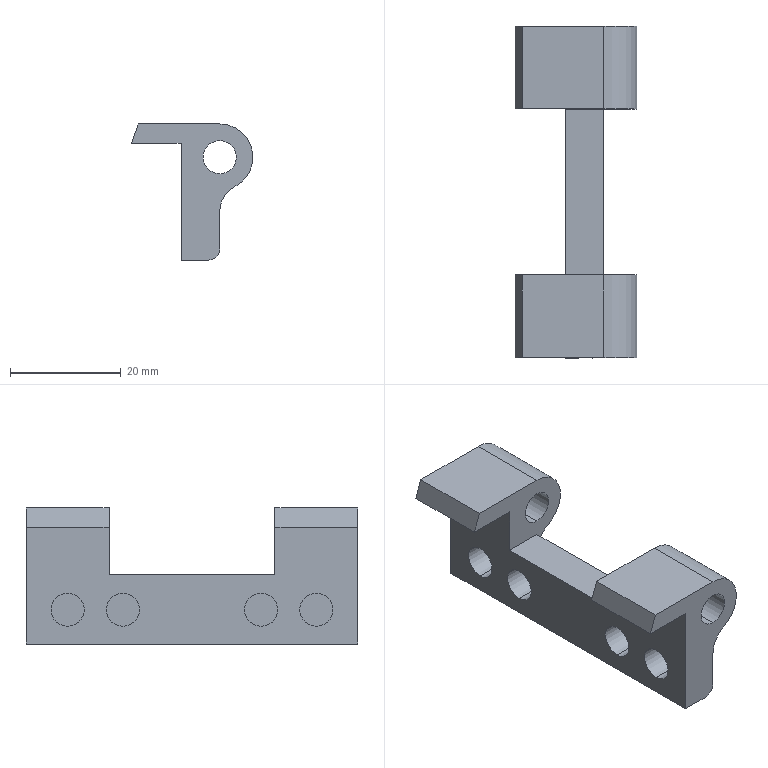Component | SolidWorks | LeftFrontDoorAssembly-1_GL213-1Hinge1-1 | 1 solid | 35 faces | box 22 x 60 x 24.6 mm | volume 8989 mm3 | plane 18 | cylinder 17 | commonest cylinder face diameters 6 x12 10 x2 12 x2 4 x1
STEP:
#1=COLOUR_RGB('',0.7922,0.8196,0.9333);
#2=FILL_AREA_STYLE_COLOUR('',#1);
#3=FILL_AREA_STYLE('',(#2));
#4=SURFACE_STYLE_FILL_AREA(#3);
#5=SURFACE_SIDE_STYLE('',(#4));
#6=SURFACE_STYLE_USAGE(.BOTH.,#5);
#7=PRESENTATION_STYLE_ASSIGNMENT((#6));
#8=CARTESIAN_POINT('',(29.637,61.402,15.142));
#9=VERTEX_POINT('',#8);
#10=CARTESIAN_POINT('',(29.637,61.402,14.906));
#11=VERTEX_POINT('',#10);
#12=CARTESIAN_POINT('',(29.637,61.402,15.024));
#13=DIRECTION('',(-1.,-0.,-0.));
#14=DIRECTION('',(0.,0.,-1.));
#15=AXIS2_PLACEMENT_3D('',#12,#13,#14);
#16=CIRCLE('',#15,0.1181);
#17=EDGE_CURVE('',#9,#11,#16,.T.);
#18=ORIENTED_EDGE('',*,*,#17,.F.);
#19=CARTESIAN_POINT('',(29.44,61.402,15.142));
#20=VERTEX_POINT('',#19);
#21=CARTESIAN_POINT('',(29.637,61.402,15.142));
#22=DIRECTION('',(-1.,-0.,-0.));
#23=VECTOR('',#22,39.37);
#24=LINE('',#21,#23);
#25=EDGE_CURVE('',#9,#20,#24,.T.);
#26=ORIENTED_EDGE('',*,*,#25,.T.);
#27=CARTESIAN_POINT('',(29.44,61.402,14.906));
#28=VERTEX_POINT('',#27);
#29=CARTESIAN_POINT('',(29.44,61.402,15.024));
#30=DIRECTION('',(-1.,-0.,-0.));
#31=DIRECTION('',(0.,0.,-1.));
#32=AXIS2_PLACEMENT_3D('',#29,#30,#31);
#33=CIRCLE('',#32,0.1181);
#34=EDGE_CURVE('',#20,#28,#33,.T.);
#35=ORIENTED_EDGE('',*,*,#34,.T.);
#36=CARTESIAN_POINT('',(29.637,61.402,14.906));
#37=DIRECTION('',(-1.,-0.,-0.));
#38=VECTOR('',#37,39.37);
#39=LINE('',#36,#38);
#40=EDGE_CURVE('',#11,#28,#39,.T.);
#41=ORIENTED_EDGE('',*,*,#40,.F.);
#42=EDGE_LOOP('',(#18,#26,#35,#41));
#43=FACE_OUTER_BOUND('',#42,.T.);
#44=CARTESIAN_POINT('',(29.637,61.402,15.024));
#45=DIRECTION('',(-1.,-0.,-0.));
#46=DIRECTION('',(0.,0.,-1.));
#47=AXIS2_PLACEMENT_3D('',#44,#45,#46);
#48=CYLINDRICAL_SURFACE('',#47,0.1181);
#49=ADVANCED_FACE('',(#43),#48,.F.);
#50=CARTESIAN_POINT('',(29.637,61.795,15.142));
#51=VERTEX_POINT('',#50);
#52=CARTESIAN_POINT('',(29.637,61.795,14.906));
#53=VERTEX_POINT('',#52);
#54=CARTESIAN_POINT('',(29.637,61.795,15.024));
#55=DIRECTION('',(-1.,-0.,-0.));
#56=DIRECTION('',(0.,0.,-1.));
#57=AXIS2_PLACEMENT_3D('',#54,#55,#56);
#58=CIRCLE('',#57,0.1181);
#59=EDGE_CURVE('',#51,#53,#58,.T.);
#60=ORIENTED_EDGE('',*,*,#59,.F.);
#61=CARTESIAN_POINT('',(29.44,61.795,15.142));
#62=VERTEX_POINT('',#61);
#63=CARTESIAN_POINT('',(29.637,61.795,15.142));
#64=DIRECTION('',(-1.,-0.,-0.));
#65=VECTOR('',#64,39.37);
#66=LINE('',#63,#65);
#67=EDGE_CURVE('',#51,#62,#66,.T.);
#68=ORIENTED_EDGE('',*,*,#67,.T.);
#69=CARTESIAN_POINT('',(29.44,61.795,14.906));
#70=VERTEX_POINT('',#69);
#71=CARTESIAN_POINT('',(29.44,61.795,15.024));
#72=DIRECTION('',(-1.,-0.,-0.));
#73=DIRECTION('',(0.,0.,-1.));
#74=AXIS2_PLACEMENT_3D('',#71,#72,#73);
#75=CIRCLE('',#74,0.1181);
#76=EDGE_CURVE('',#62,#70,#75,.T.);
#77=ORIENTED_EDGE('',*,*,#76,.T.);
#78=CARTESIAN_POINT('',(29.637,61.795,14.906));
#79=DIRECTION('',(-1.,-0.,-0.));
#80=VECTOR('',#79,39.37);
#81=LINE('',#78,#80);
#82=EDGE_CURVE('',#53,#70,#81,.T.);
#83=ORIENTED_EDGE('',*,*,#82,.F.);
#84=EDGE_LOOP('',(#60,#68,#77,#83));
#85=FACE_OUTER_BOUND('',#84,.T.);
#86=CARTESIAN_POINT('',(29.637,61.795,15.024));
#87=DIRECTION('',(-1.,-0.,-0.));
#88=DIRECTION('',(0.,0.,-1.));
#89=AXIS2_PLACEMENT_3D('',#86,#87,#88);
#90=CYLINDRICAL_SURFACE('',#89,0.1181);
#91=ADVANCED_FACE('',(#85),#90,.F.);
#92=CARTESIAN_POINT('',(29.637,62.78,15.142));
#93=VERTEX_POINT('',#92);
#94=CARTESIAN_POINT('',(29.637,62.78,14.906));
#95=VERTEX_POINT('',#94);
#96=CARTESIAN_POINT('',(29.637,62.78,15.024));
#97=DIRECTION('',(-1.,-0.,-0.));
#98=DIRECTION('',(0.,0.,-1.));
#99=AXIS2_PLACEMENT_3D('',#96,#97,#98);
#100=CIRCLE('',#99,0.1181);
#101=EDGE_CURVE('',#93,#95,#100,.T.);
#102=ORIENTED_EDGE('',*,*,#101,.F.);
#103=CARTESIAN_POINT('',(29.44,62.78,15.142));
#104=VERTEX_POINT('',#103);
#105=CARTESIAN_POINT('',(29.637,62.78,15.142));
#106=DIRECTION('',(-1.,-0.,-0.));
#107=VECTOR('',#106,39.37);
#108=LINE('',#105,#107);
#109=EDGE_CURVE('',#93,#104,#108,.T.);
#110=ORIENTED_EDGE('',*,*,#109,.T.);
#111=CARTESIAN_POINT('',(29.44,62.78,14.906));
#112=VERTEX_POINT('',#111);
#113=CARTESIAN_POINT('',(29.44,62.78,15.024));
#114=DIRECTION('',(-1.,-0.,-0.));
#115=DIRECTION('',(0.,0.,-1.));
#116=AXIS2_PLACEMENT_3D('',#113,#114,#115);
#117=CIRCLE('',#116,0.1181);
#118=EDGE_CURVE('',#104,#112,#117,.T.);
#119=ORIENTED_EDGE('',*,*,#118,.T.);
#120=CARTESIAN_POINT('',(29.637,62.78,14.906));
#121=DIRECTION('',(-1.,-0.,-0.));
#122=VECTOR('',#121,39.37);
#123=LINE('',#120,#122);
#124=EDGE_CURVE('',#95,#112,#123,.T.);
#125=ORIENTED_EDGE('',*,*,#124,.F.);
#126=EDGE_LOOP('',(#102,#110,#119,#125));
#127=FACE_OUTER_BOUND('',#126,.T.);
#128=CARTESIAN_POINT('',(29.637,62.78,15.024));
#129=DIRECTION('',(-1.,-0.,-0.));
#130=DIRECTION('',(0.,0.,-1.));
#131=AXIS2_PLACEMENT_3D('',#128,#129,#130);
#132=CYLINDRICAL_SURFACE('',#131,0.1181);
#133=ADVANCED_FACE('',(#127),#132,.F.);
#134=CARTESIAN_POINT('',(29.637,63.173,15.142));
#135=VERTEX_POINT('',#134);
#136=CARTESIAN_POINT('',(29.637,63.173,14.906));
#137=VERTEX_POINT('',#136);
#138=CARTESIAN_POINT('',(29.637,63.173,15.024));
#139=DIRECTION('',(-1.,-0.,-0.));
#140=DIRECTION('',(0.,0.,-1.));
#141=AXIS2_PLACEMENT_3D('',#138,#139,#140);
#142=CIRCLE('',#141,0.1181);
#143=EDGE_CURVE('',#135,#137,#142,.T.);
#144=ORIENTED_EDGE('',*,*,#143,.F.);
#145=CARTESIAN_POINT('',(29.44,63.173,15.142));
#146=VERTEX_POINT('',#145);
#147=CARTESIAN_POINT('',(29.637,63.173,15.142));
#148=DIRECTION('',(-1.,-0.,-0.));
#149=VECTOR('',#148,39.37);
#150=LINE('',#147,#149);
#151=EDGE_CURVE('',#135,#146,#150,.T.);
#152=ORIENTED_EDGE('',*,*,#151,.T.);
#153=CARTESIAN_POINT('',(29.44,63.173,14.906));
#154=VERTEX_POINT('',#153);
#155=CARTESIAN_POINT('',(29.44,63.173,15.024));
#156=DIRECTION('',(-1.,-0.,-0.));
#157=DIRECTION('',(0.,0.,-1.));
#158=AXIS2_PLACEMENT_3D('',#155,#156,#157);
#159=CIRCLE('',#158,0.1181);
#160=EDGE_CURVE('',#146,#154,#159,.T.);
#161=ORIENTED_EDGE('',*,*,#160,.T.);
#162=CARTESIAN_POINT('',(29.637,63.173,14.906));
#163=DIRECTION('',(-1.,-0.,-0.));
#164=VECTOR('',#163,39.37);
#165=LINE('',#162,#164);
#166=EDGE_CURVE('',#137,#154,#165,.T.);
#167=ORIENTED_EDGE('',*,*,#166,.F.);
#168=EDGE_LOOP('',(#144,#152,#161,#167));
#169=FACE_OUTER_BOUND('',#168,.T.);
#170=CARTESIAN_POINT('',(29.637,63.173,15.024));
#171=DIRECTION('',(-1.,-0.,-0.));
#172=DIRECTION('',(0.,0.,-1.));
#173=AXIS2_PLACEMENT_3D('',#170,#171,#172);
#174=CYLINDRICAL_SURFACE('',#173,0.1181);
#175=ADVANCED_FACE('',(#169),#174,.F.);
#176=CARTESIAN_POINT('',(29.716,63.468,15.63));
#177=VERTEX_POINT('',#176);
#178=CARTESIAN_POINT('',(29.716,63.468,15.394));
#179=VERTEX_POINT('',#178);
#180=CARTESIAN_POINT('',(29.716,63.468,15.512));
#181=DIRECTION('',(0.,-1.,0.));
#182=DIRECTION('',(0.,0.,-1.));
#183=AXIS2_PLACEMENT_3D('',#180,#181,#182);
#184=CIRCLE('',#183,0.1181);
#185=EDGE_CURVE('',#177,#179,#184,.T.);
#186=ORIENTED_EDGE('',*,*,#185,.F.);
#187=CARTESIAN_POINT('',(29.716,62.878,15.63));
#188=VERTEX_POINT('',#187);
#189=CARTESIAN_POINT('',(29.716,63.468,15.63));
#190=DIRECTION('',(0.,-1.,0.));
#191=VECTOR('',#190,39.37);
#192=LINE('',#189,#191);
#193=EDGE_CURVE('',#177,#188,#192,.T.);
#194=ORIENTED_EDGE('',*,*,#193,.T.);
#195=CARTESIAN_POINT('',(29.716,62.878,15.394));
#196=VERTEX_POINT('',#195);
#197=CARTESIAN_POINT('',(29.716,62.878,15.512));
#198=DIRECTION('',(-0.,1.,-0.));
#199=DIRECTION('',(0.,0.,-1.));
#200=AXIS2_PLACEMENT_3D('',#197,#198,#199);
#201=CIRCLE('',#200,0.1181);
#202=EDGE_CURVE('',#196,#188,#201,.T.);
#203=ORIENTED_EDGE('',*,*,#202,.F.);
#204=CARTESIAN_POINT('',(29.716,63.468,15.394));
#205=DIRECTION('',(0.,-1.,0.));
#206=VECTOR('',#205,39.37);
#207=LINE('',#204,#206);
#208=EDGE_CURVE('',#179,#196,#207,.T.);
#209=ORIENTED_EDGE('',*,*,#208,.F.);
#210=EDGE_LOOP('',(#186,#194,#203,#209));
#211=FACE_OUTER_BOUND('',#210,.T.);
#212=CARTESIAN_POINT('',(29.716,63.468,15.512));
#213=DIRECTION('',(0.,-1.,0.));
#214=DIRECTION('',(0.,0.,-1.));
#215=AXIS2_PLACEMENT_3D('',#212,#213,#214);
#216=CYLINDRICAL_SURFACE('',#215,0.1181);
#217=ADVANCED_FACE('',(#211),#216,.F.);
#218=CARTESIAN_POINT('',(29.716,61.697,15.63));
#219=VERTEX_POINT('',#218);
#220=CARTESIAN_POINT('',(29.716,61.697,15.394));
#221=VERTEX_POINT('',#220);
#222=CARTESIAN_POINT('',(29.716,61.697,15.512));
#223=DIRECTION('',(0.,-1.,0.));
#224=DIRECTION('',(-0.,0.,1.));
#225=AXIS2_PLACEMENT_3D('',#222,#223,#224);
#226=CIRCLE('',#225,0.1181);
#227=EDGE_CURVE('',#219,#221,#226,.T.);
#228=ORIENTED_EDGE('',*,*,#227,.F.);
#229=CARTESIAN_POINT('',(29.716,61.106,15.63));
#230=VERTEX_POINT('',#229);
#231=CARTESIAN_POINT('',(29.716,63.468,15.63));
#232=DIRECTION('',(0.,-1.,0.));
#233=VECTOR('',#232,39.37);
#234=LINE('',#231,#233);
#235=EDGE_CURVE('',#219,#230,#234,.T.);
#236=ORIENTED_EDGE('',*,*,#235,.T.);
#237=CARTESIAN_POINT('',(29.716,61.106,15.394));
#238=VERTEX_POINT('',#237);
#239=CARTESIAN_POINT('',(29.716,61.106,15.512));
#240=DIRECTION('',(0.,-1.,0.));
#241=DIRECTION('',(0.,0.,-1.));
#242=AXIS2_PLACEMENT_3D('',#239,#240,#241);
#243=CIRCLE('',#242,0.1181);
#244=EDGE_CURVE('',#230,#238,#243,.T.);
#245=ORIENTED_EDGE('',*,*,#244,.T.);
#246=CARTESIAN_POINT('',(29.716,63.468,15.394));
#247=DIRECTION('',(0.,-1.,0.));
#248=VECTOR('',#247,39.37);
#249=LINE('',#246,#248);
#250=EDGE_CURVE('',#221,#238,#249,.T.);
#251=ORIENTED_EDGE('',*,*,#250,.F.);
#252=EDGE_LOOP('',(#228,#236,#245,#251));
#253=FACE_OUTER_BOUND('',#252,.T.);
#254=CARTESIAN_POINT('',(29.716,63.468,15.512));
#255=DIRECTION('',(0.,-1.,0.));
#256=DIRECTION('',(0.,0.,-1.));
#257=AXIS2_PLACEMENT_3D('',#254,#255,#256);
#258=CYLINDRICAL_SURFACE('',#257,0.1181);
#259=ADVANCED_FACE('',(#253),#258,.F.);
#260=CARTESIAN_POINT('',(29.716,61.106,15.126));
#261=VERTEX_POINT('',#260);
#262=CARTESIAN_POINT('',(29.716,61.697,15.126));
#263=VERTEX_POINT('',#262);
#264=CARTESIAN_POINT('',(29.716,61.106,15.126));
#265=DIRECTION('',(-0.,1.,-0.));
#266=VECTOR('',#265,39.37);
#267=LINE('',#264,#266);
#268=EDGE_CURVE('',#261,#263,#267,.T.);
#269=ORIENTED_EDGE('',*,*,#268,.T.);
#270=CARTESIAN_POINT('',(29.823,61.697,15.301));
#271=VERTEX_POINT('',#270);
#272=CARTESIAN_POINT('',(29.913,61.697,15.126));
#273=DIRECTION('',(0.,-1.,0.));
#274=DIRECTION('',(-0.,0.,1.));
#275=AXIS2_PLACEMENT_3D('',#272,#273,#274);
#276=CIRCLE('',#275,0.1969);
#277=EDGE_CURVE('',#271,#263,#276,.T.);
#278=ORIENTED_EDGE('',*,*,#277,.F.);
#279=CARTESIAN_POINT('',(29.823,61.106,15.301));
#280=VERTEX_POINT('',#279);
#281=CARTESIAN_POINT('',(29.823,61.106,15.301));
#282=DIRECTION('',(-0.,1.,-0.));
#283=VECTOR('',#282,39.37);
#284=LINE('',#281,#283);
#285=EDGE_CURVE('',#280,#271,#284,.T.);
#286=ORIENTED_EDGE('',*,*,#285,.F.);
#287=CARTESIAN_POINT('',(29.913,61.106,15.126));
#288=DIRECTION('',(-0.,1.,-0.));
#289=DIRECTION('',(0.,0.,-1.));
#290=AXIS2_PLACEMENT_3D('',#287,#288,#289);
#291=CIRCLE('',#290,0.1969);
#292=EDGE_CURVE('',#261,#280,#291,.T.);
#293=ORIENTED_EDGE('',*,*,#292,.F.);
#294=EDGE_LOOP('',(#269,#278,#286,#293));
#295=FACE_OUTER_BOUND('',#294,.T.);
#296=CARTESIAN_POINT('',(29.913,61.106,15.126));
#297=DIRECTION('',(-0.,1.,-0.));
#298=DIRECTION('',(-0.,0.,1.));
#299=AXIS2_PLACEMENT_3D('',#296,#297,#298);
#300=CYLINDRICAL_SURFACE('',#299,0.1969);
#301=ADVANCED_FACE('',(#295),#300,.F.);
#302=CARTESIAN_POINT('',(29.716,62.878,15.126));
#303=VERTEX_POINT('',#302);
#304=CARTESIAN_POINT('',(29.823,62.878,15.301));
#305=VERTEX_POINT('',#304);
#306=CARTESIAN_POINT('',(29.913,62.878,15.126));
#307=DIRECTION('',(-0.,1.,-0.));
#308=DIRECTION('',(0.,0.,-1.));
#309=AXIS2_PLACEMENT_3D('',#306,#307,#308);
#310=CIRCLE('',#309,0.1969);
#311=EDGE_CURVE('',#303,#305,#310,.T.);
#312=ORIENTED_EDGE('',*,*,#311,.F.);
#313=CARTESIAN_POINT('',(29.716,63.468,15.126));
#314=VERTEX_POINT('',#313);
#315=CARTESIAN_POINT('',(29.716,61.106,15.126));
#316=DIRECTION('',(-0.,1.,-0.));
#317=VECTOR('',#316,39.37);
#318=LINE('',#315,#317);
#319=EDGE_CURVE('',#303,#314,#318,.T.);
#320=ORIENTED_EDGE('',*,*,#319,.T.);
#321=CARTESIAN_POINT('',(29.823,63.468,15.301));
#322=VERTEX_POINT('',#321);
#323=CARTESIAN_POINT('',(29.913,63.468,15.126));
#324=DIRECTION('',(-0.,1.,-0.));
#325=DIRECTION('',(0.,0.,-1.));
#326=AXIS2_PLACEMENT_3D('',#323,#324,#325);
#327=CIRCLE('',#326,0.1969);
#328=EDGE_CURVE('',#314,#322,#327,.T.);
#329=ORIENTED_EDGE('',*,*,#328,.T.);
#330=CARTESIAN_POINT('',(29.823,61.106,15.301));
#331=DIRECTION('',(-0.,1.,-0.));
#332=VECTOR('',#331,39.37);
#333=LINE('',#330,#332);
#334=EDGE_CURVE('',#305,#322,#333,.T.);
#335=ORIENTED_EDGE('',*,*,#334,.F.);
#336=EDGE_LOOP('',(#312,#320,#329,#335));
#337=FACE_OUTER_BOUND('',#336,.T.);
#338=CARTESIAN_POINT('',(29.913,61.106,15.126));
#339=DIRECTION('',(-0.,1.,-0.));
#340=DIRECTION('',(-0.,0.,1.));
#341=AXIS2_PLACEMENT_3D('',#338,#339,#340);
#342=CYLINDRICAL_SURFACE('',#341,0.1969);
#343=ADVANCED_FACE('',(#337),#342,.F.);
#344=CARTESIAN_POINT('',(29.716,61.697,15.276));
#345=VERTEX_POINT('',#344);
#346=CARTESIAN_POINT('',(29.44,61.697,15.276));
#347=VERTEX_POINT('',#346);
#348=CARTESIAN_POINT('',(32.078,61.697,15.276));
#349=DIRECTION('',(-1.,-0.,-0.));
#350=VECTOR('',#349,39.37);
#351=LINE('',#348,#350);
#352=EDGE_CURVE('',#345,#347,#351,.T.);
#353=ORIENTED_EDGE('',*,*,#352,.F.);
#354=CARTESIAN_POINT('',(29.716,62.878,15.276));
#355=VERTEX_POINT('',#354);
#356=CARTESIAN_POINT('',(29.716,62.878,15.276));
#357=DIRECTION('',(0.,-1.,0.));
#358=VECTOR('',#357,39.37);
#359=LINE('',#356,#358);
#360=EDGE_CURVE('',#355,#345,#359,.T.);
#361=ORIENTED_EDGE('',*,*,#360,.F.);
#362=CARTESIAN_POINT('',(29.44,62.878,15.276));
#363=VERTEX_POINT('',#362);
#364=CARTESIAN_POINT('',(32.078,62.878,15.276));
#365=DIRECTION('',(-1.,-0.,-0.));
#366=VECTOR('',#365,39.37);
#367=LINE('',#364,#366);
#368=EDGE_CURVE('',#355,#363,#367,.T.);
#369=ORIENTED_EDGE('',*,*,#368,.T.);
#370=CARTESIAN_POINT('',(29.44,61.106,15.276));
#371=DIRECTION('',(0.,-1.,0.));
#372=VECTOR('',#371,39.37);
#373=LINE('',#370,#372);
#374=EDGE_CURVE('',#363,#347,#373,.T.);
#375=ORIENTED_EDGE('',*,*,#374,.T.);
#376=EDGE_LOOP('',(#353,#361,#369,#375));
#377=FACE_OUTER_BOUND('',#376,.T.);
#378=CARTESIAN_POINT('',(32.078,62.878,15.276));
#379=DIRECTION('',(-0.,0.,1.));
#380=DIRECTION('',(-1.,-0.,-0.));
#381=AXIS2_PLACEMENT_3D('',#378,#379,#380);
#382=PLANE('',#381);
#383=ADVANCED_FACE('',(#377),#382,.T.);
#384=CARTESIAN_POINT('',(29.44,61.697,15.61));
#385=VERTEX_POINT('',#384);
#386=CARTESIAN_POINT('',(29.086,61.697,15.61));
#387=VERTEX_POINT('',#386);
#388=CARTESIAN_POINT('',(29.44,61.697,15.61));
#389=DIRECTION('',(-1.,-0.,-0.));
#390=VECTOR('',#389,39.37);
#391=LINE('',#388,#390);
#392=EDGE_CURVE('',#385,#387,#391,.T.);
#393=ORIENTED_EDGE('',*,*,#392,.F.);
#394=CARTESIAN_POINT('',(29.44,61.106,15.61));
#395=VERTEX_POINT('',#394);
#396=CARTESIAN_POINT('',(29.44,61.106,15.61));
#397=DIRECTION('',(-0.,1.,-0.));
#398=VECTOR('',#397,39.37);
#399=LINE('',#396,#398);
#400=EDGE_CURVE('',#395,#385,#399,.T.);
#401=ORIENTED_EDGE('',*,*,#400,.F.);
#402=CARTESIAN_POINT('',(29.086,61.106,15.61));
#403=VERTEX_POINT('',#402);
#404=CARTESIAN_POINT('',(29.44,61.106,15.61));
#405=DIRECTION('',(1.,0.,0.));
#406=VECTOR('',#405,39.37);
#407=LINE('',#404,#406);
#408=EDGE_CURVE('',#403,#395,#407,.T.);
#409=ORIENTED_EDGE('',*,*,#408,.F.);
#410=CARTESIAN_POINT('',(29.086,61.106,15.61));
#411=DIRECTION('',(-0.,1.,-0.));
#412=VECTOR('',#411,39.37);
#413=LINE('',#410,#412);
#414=EDGE_CURVE('',#403,#387,#413,.T.);
#415=ORIENTED_EDGE('',*,*,#414,.T.);
#416=EDGE_LOOP('',(#393,#401,#409,#415));
#417=FACE_OUTER_BOUND('',#416,.T.);
#418=CARTESIAN_POINT('',(29.44,61.106,15.61));
#419=DIRECTION('',(-0.,0.,1.));
#420=DIRECTION('',(-1.,-0.,-0.));
#421=AXIS2_PLACEMENT_3D('',#418,#419,#420);
#422=PLANE('',#421);
#423=ADVANCED_FACE('',(#417),#422,.F.);
#424=CARTESIAN_POINT('',(29.086,62.878,15.61));
#425=VERTEX_POINT('',#424);
#426=CARTESIAN_POINT('',(29.44,62.878,15.61));
#427=VERTEX_POINT('',#426);
#428=CARTESIAN_POINT('',(29.44,62.878,15.61));
#429=DIRECTION('',(1.,0.,0.));
#430=VECTOR('',#429,39.37);
#431=LINE('',#428,#430);
#432=EDGE_CURVE('',#425,#427,#431,.T.);
#433=ORIENTED_EDGE('',*,*,#432,.F.);
#434=CARTESIAN_POINT('',(29.086,63.468,15.61));
#435=VERTEX_POINT('',#434);
#436=CARTESIAN_POINT('',(29.086,61.106,15.61));
#437=DIRECTION('',(-0.,1.,-0.));
#438=VECTOR('',#437,39.37);
#439=LINE('',#436,#438);
#440=EDGE_CURVE('',#425,#435,#439,.T.);
#441=ORIENTED_EDGE('',*,*,#440,.T.);
#442=CARTESIAN_POINT('',(29.44,63.468,15.61));
#443=VERTEX_POINT('',#442);
#444=CARTESIAN_POINT('',(29.44,63.468,15.61));
#445=DIRECTION('',(1.,0.,0.));
#446=VECTOR('',#445,39.37);
#447=LINE('',#444,#446);
#448=EDGE_CURVE('',#435,#443,#447,.T.);
#449=ORIENTED_EDGE('',*,*,#448,.T.);
#450=CARTESIAN_POINT('',(29.44,61.106,15.61));
#451=DIRECTION('',(-0.,1.,-0.));
#452=VECTOR('',#451,39.37);
#453=LINE('',#450,#452);
#454=EDGE_CURVE('',#427,#443,#453,.T.);
#455=ORIENTED_EDGE('',*,*,#454,.F.);
#456=EDGE_LOOP('',(#433,#441,#449,#455));
#457=FACE_OUTER_BOUND('',#456,.T.);
#458=CARTESIAN_POINT('',(29.44,61.106,15.61));
#459=DIRECTION('',(-0.,0.,1.));
#460=DIRECTION('',(-1.,-0.,-0.));
#461=AXIS2_PLACEMENT_3D('',#458,#459,#460);
#462=PLANE('',#461);
#463=ADVANCED_FACE('',(#457),#462,.F.);
#464=CARTESIAN_POINT('',(29.44,61.402,15.024));
#465=DIRECTION('',(-1.,-0.,-0.));
#466=DIRECTION('',(0.,0.,-1.));
#467=AXIS2_PLACEMENT_3D('',#464,#465,#466);
#468=CIRCLE('',#467,0.1181);
#469=EDGE_CURVE('',#28,#20,#468,.T.);
#470=ORIENTED_EDGE('',*,*,#469,.F.);
#471=ORIENTED_EDGE('',*,*,#34,.F.);
#472=EDGE_LOOP('',(#470,#471));
#473=FACE_BOUND('',#472,.T.);
#474=CARTESIAN_POINT('',(29.44,61.795,15.024));
#475=DIRECTION('',(-1.,-0.,-0.));
#476=DIRECTION('',(0.,0.,-1.));
#477=AXIS2_PLACEMENT_3D('',#474,#475,#476);
#478=CIRCLE('',#477,0.1181);
#479=EDGE_CURVE('',#70,#62,#478,.T.);
#480=ORIENTED_EDGE('',*,*,#479,.F.);
#481=ORIENTED_EDGE('',*,*,#76,.F.);
#482=EDGE_LOOP('',(#480,#481));
#483=FACE_BOUND('',#482,.T.);
#484=CARTESIAN_POINT('',(29.44,62.78,15.024));
#485=DIRECTION('',(-1.,-0.,-0.));
#486=DIRECTION('',(0.,0.,-1.));
#487=AXIS2_PLACEMENT_3D('',#484,#485,#486);
#488=CIRCLE('',#487,0.1181);
#489=EDGE_CURVE('',#112,#104,#488,.T.);
#490=ORIENTED_EDGE('',*,*,#489,.F.);
#491=ORIENTED_EDGE('',*,*,#118,.F.);
#492=EDGE_LOOP('',(#490,#491));
#493=FACE_BOUND('',#492,.T.);
#494=CARTESIAN_POINT('',(29.44,63.173,15.024));
#495=DIRECTION('',(-1.,-0.,-0.));
#496=DIRECTION('',(0.,0.,-1.));
#497=AXIS2_PLACEMENT_3D('',#494,#495,#496);
#498=CIRCLE('',#497,0.1181);
#499=EDGE_CURVE('',#154,#146,#498,.T.);
#500=ORIENTED_EDGE('',*,*,#499,.F.);
#501=ORIENTED_EDGE('',*,*,#160,.F.);
#502=EDGE_LOOP('',(#500,#501));
#503=FACE_BOUND('',#502,.T.);
#504=CARTESIAN_POINT('',(29.44,61.697,14.78));
#505=DIRECTION('',(-0.,0.,1.));
#506=VECTOR('',#505,39.37);
#507=LINE('',#504,#506);
#508=EDGE_CURVE('',#347,#385,#507,.T.);
#509=ORIENTED_EDGE('',*,*,#508,.F.);
#510=ORIENTED_EDGE('',*,*,#374,.F.);
#511=CARTESIAN_POINT('',(29.44,62.878,14.78));
#512=DIRECTION('',(0.,-0.,-1.));
#513=VECTOR('',#512,39.37);
#514=LINE('',#511,#513);
#515=EDGE_CURVE('',#427,#363,#514,.T.);
#516=ORIENTED_EDGE('',*,*,#515,.F.);
#517=ORIENTED_EDGE('',*,*,#454,.T.);
#518=CARTESIAN_POINT('',(29.44,63.468,14.78));
#519=VERTEX_POINT('',#518);
#520=CARTESIAN_POINT('',(29.44,63.468,14.78));
#521=DIRECTION('',(0.,-0.,-1.));
#522=VECTOR('',#521,39.37);
#523=LINE('',#520,#522);
#524=EDGE_CURVE('',#443,#519,#523,.T.);
#525=ORIENTED_EDGE('',*,*,#524,.T.);
#526=CARTESIAN_POINT('',(29.44,61.106,14.78));
#527=VERTEX_POINT('',#526);
#528=CARTESIAN_POINT('',(29.44,61.106,14.78));
#529=DIRECTION('',(-0.,1.,-0.));
#530=VECTOR('',#529,39.37);
#531=LINE('',#528,#530);
#532=EDGE_CURVE('',#527,#519,#531,.T.);
#533=ORIENTED_EDGE('',*,*,#532,.F.);
#534=CARTESIAN_POINT('',(29.44,61.106,14.78));
#535=DIRECTION('',(0.,-0.,-1.));
#536=VECTOR('',#535,39.37);
#537=LINE('',#534,#536);
#538=EDGE_CURVE('',#395,#527,#537,.T.);
#539=ORIENTED_EDGE('',*,*,#538,.F.);
#540=ORIENTED_EDGE('',*,*,#400,.T.);
#541=EDGE_LOOP('',(#509,#510,#516,#517,#525,#533,#539,#540));
#542=FACE_OUTER_BOUND('',#541,.T.);
#543=CARTESIAN_POINT('',(29.44,61.106,14.78));
#544=DIRECTION('',(1.,0.,0.));
#545=DIRECTION('',(-0.,0.,1.));
#546=AXIS2_PLACEMENT_3D('',#543,#544,#545);
#547=PLANE('',#546);
#548=ADVANCED_FACE('',(#473,#483,#493,#503,#542),#547,.F.);
#549=CARTESIAN_POINT('',(29.716,61.697,15.748));
#550=VERTEX_POINT('',#549);
#551=CARTESIAN_POINT('',(29.716,61.697,15.512));
#552=DIRECTION('',(-0.,1.,-0.));
#553=DIRECTION('',(-0.,0.,1.));
#554=AXIS2_PLACEMENT_3D('',#551,#552,#553);
#555=CIRCLE('',#554,0.2362);
#556=EDGE_CURVE('',#550,#271,#555,.T.);
#557=ORIENTED_EDGE('',*,*,#556,.F.);
#558=CARTESIAN_POINT('',(29.716,61.106,15.748));
#559=VERTEX_POINT('',#558);
#560=CARTESIAN_POINT('',(29.716,61.106,15.748));
#561=DIRECTION('',(-0.,1.,-0.));
#562=VECTOR('',#561,39.37);
#563=LINE('',#560,#562);
#564=EDGE_CURVE('',#559,#550,#563,.T.);
#565=ORIENTED_EDGE('',*,*,#564,.F.);
#566=CARTESIAN_POINT('',(29.716,61.106,15.512));
#567=DIRECTION('',(0.,-1.,0.));
#568=DIRECTION('',(-0.,0.,1.));
#569=AXIS2_PLACEMENT_3D('',#566,#567,#568);
#570=CIRCLE('',#569,0.2362);
#571=EDGE_CURVE('',#280,#559,#570,.T.);
#572=ORIENTED_EDGE('',*,*,#571,.F.);
#573=ORIENTED_EDGE('',*,*,#285,.T.);
#574=EDGE_LOOP('',(#557,#565,#572,#573));
#575=FACE_OUTER_BOUND('',#574,.T.);
#576=CARTESIAN_POINT('',(29.716,61.106,15.512));
#577=DIRECTION('',(-0.,1.,-0.));
#578=DIRECTION('',(-0.,0.,1.));
#579=AXIS2_PLACEMENT_3D('',#576,#577,#578);
#580=CYLINDRICAL_SURFACE('',#579,0.2362);
#581=ADVANCED_FACE('',(#575),#580,.T.);
#582=CARTESIAN_POINT('',(29.716,62.878,15.748));
#583=VERTEX_POINT('',#582);
#584=CARTESIAN_POINT('',(29.716,62.878,15.512));
#585=DIRECTION('',(0.,-1.,0.));
#586=DIRECTION('',(0.,0.,-1.));
#587=AXIS2_PLACEMENT_3D('',#584,#585,#586);
#588=CIRCLE('',#587,0.2362);
#589=EDGE_CURVE('',#305,#583,#588,.T.);
#590=ORIENTED_EDGE('',*,*,#589,.F.);
#591=ORIENTED_EDGE('',*,*,#334,.T.);
#592=CARTESIAN_POINT('',(29.716,63.468,15.748));
#593=VERTEX_POINT('',#592);
#594=CARTESIAN_POINT('',(29.716,63.468,15.512));
#595=DIRECTION('',(0.,-1.,0.));
#596=DIRECTION('',(-0.,0.,1.));
#597=AXIS2_PLACEMENT_3D('',#594,#595,#596);
#598=CIRCLE('',#597,0.2362);
#599=EDGE_CURVE('',#322,#593,#598,.T.);
#600=ORIENTED_EDGE('',*,*,#599,.T.);
#601=CARTESIAN_POINT('',(29.716,61.106,15.748));
#602=DIRECTION('',(-0.,1.,-0.));
#603=VECTOR('',#602,39.37);
#604=LINE('',#601,#603);
#605=EDGE_CURVE('',#583,#593,#604,.T.);
#606=ORIENTED_EDGE('',*,*,#605,.F.);
#607=EDGE_LOOP('',(#590,#591,#600,#606));
#608=FACE_OUTER_BOUND('',#607,.T.);
#609=CARTESIAN_POINT('',(29.716,61.106,15.512));
#610=DIRECTION('',(-0.,1.,-0.));
#611=DIRECTION('',(-0.,0.,1.));
#612=AXIS2_PLACEMENT_3D('',#609,#610,#611);
#613=CYLINDRICAL_SURFACE('',#612,0.2362);
#614=ADVANCED_FACE('',(#608),#613,.T.);
#615=CARTESIAN_POINT('',(29.136,61.697,15.748));
#616=VERTEX_POINT('',#615);
#617=CARTESIAN_POINT('',(32.078,61.697,15.748));
#618=DIRECTION('',(-1.,-0.,-0.));
#619=VECTOR('',#618,39.37);
#620=LINE('',#617,#619);
#621=EDGE_CURVE('',#550,#616,#620,.T.);
#622=ORIENTED_EDGE('',*,*,#621,.T.);
#623=CARTESIAN_POINT('',(29.136,61.106,15.748));
#624=VERTEX_POINT('',#623);
#625=CARTESIAN_POINT('',(29.136,63.468,15.748));
#626=DIRECTION('',(0.,-1.,0.));
#627=VECTOR('',#626,39.37);
#628=LINE('',#625,#627);
#629=EDGE_CURVE('',#616,#624,#628,.T.);
#630=ORIENTED_EDGE('',*,*,#629,.T.);
#631=CARTESIAN_POINT('',(29.086,61.106,15.748));
#632=DIRECTION('',(-1.,-0.,-0.));
#633=VECTOR('',#632,39.37);
#634=LINE('',#631,#633);
#635=EDGE_CURVE('',#559,#624,#634,.T.);
#636=ORIENTED_EDGE('',*,*,#635,.F.);
#637=ORIENTED_EDGE('',*,*,#564,.T.);
#638=EDGE_LOOP('',(#622,#630,#636,#637));
#639=FACE_OUTER_BOUND('',#638,.T.);
#640=CARTESIAN_POINT('',(29.086,61.106,15.748));
#641=DIRECTION('',(0.,-0.,-1.));
#642=DIRECTION('',(-0.,1.,-0.));
#643=AXIS2_PLACEMENT_3D('',#640,#641,#642);
#644=PLANE('',#643);
#645=ADVANCED_FACE('',(#639),#644,.F.);
#646=CARTESIAN_POINT('',(29.136,62.878,15.748));
#647=VERTEX_POINT('',#646);
#648=CARTESIAN_POINT('',(32.078,62.878,15.748));
#649=DIRECTION('',(-1.,-0.,-0.));
#650=VECTOR('',#649,39.37);
#651=LINE('',#648,#650);
#652=EDGE_CURVE('',#583,#647,#651,.T.);
#653=ORIENTED_EDGE('',*,*,#652,.F.);
#654=ORIENTED_EDGE('',*,*,#605,.T.);
#655=CARTESIAN_POINT('',(29.136,63.468,15.748));
#656=VERTEX_POINT('',#655);
#657=CARTESIAN_POINT('',(29.086,63.468,15.748));
#658=DIRECTION('',(-1.,-0.,-0.));
#659=VECTOR('',#658,39.37);
#660=LINE('',#657,#659);
#661=EDGE_CURVE('',#593,#656,#660,.T.);
#662=ORIENTED_EDGE('',*,*,#661,.T.);
#663=CARTESIAN_POINT('',(29.136,63.468,15.748));
#664=DIRECTION('',(0.,-1.,0.));
#665=VECTOR('',#664,39.37);
#666=LINE('',#663,#665);
#667=EDGE_CURVE('',#656,#647,#666,.T.);
#668=ORIENTED_EDGE('',*,*,#667,.T.);
#669=EDGE_LOOP('',(#653,#654,#662,#668));
#670=FACE_OUTER_BOUND('',#669,.T.);
#671=CARTESIAN_POINT('',(29.086,61.106,15.748));
#672=DIRECTION('',(0.,-0.,-1.));
#673=DIRECTION('',(-0.,1.,-0.));
#674=AXIS2_PLACEMENT_3D('',#671,#672,#673);
#675=PLANE('',#674);
#676=ADVANCED_FACE('',(#670),#675,.F.);
#677=CARTESIAN_POINT('',(29.086,61.697,15.61));
#678=DIRECTION('',(0.342,0.,0.9397));
#679=VECTOR('',#678,39.37);
#680=LINE('',#677,#679);
#681=EDGE_CURVE('',#387,#616,#680,.T.);
#682=ORIENTED_EDGE('',*,*,#681,.F.);
#683=ORIENTED_EDGE('',*,*,#414,.F.);
#684=CARTESIAN_POINT('',(29.086,61.106,15.61));
#685=DIRECTION('',(0.342,0.,0.9397));
#686=VECTOR('',#685,39.37);
#687=LINE('',#684,#686);
#688=EDGE_CURVE('',#403,#624,#687,.T.);
#689=ORIENTED_EDGE('',*,*,#688,.T.);
#690=ORIENTED_EDGE('',*,*,#629,.F.);
#691=EDGE_LOOP('',(#682,#683,#689,#690));
#692=FACE_OUTER_BOUND('',#691,.T.);
#693=CARTESIAN_POINT('',(29.086,63.468,15.61));
#694=DIRECTION('',(0.9397,-0.,-0.342));
#695=DIRECTION('',(0.342,0.,0.9397));
#696=AXIS2_PLACEMENT_3D('',#693,#694,#695);
#697=PLANE('',#696);
#698=ADVANCED_FACE('',(#692),#697,.F.);
#699=CARTESIAN_POINT('',(29.086,62.878,15.61));
#700=DIRECTION('',(-0.342,-0.,-0.9397));
#701=VECTOR('',#700,39.37);
#702=LINE('',#699,#701);
#703=EDGE_CURVE('',#647,#425,#702,.T.);
#704=ORIENTED_EDGE('',*,*,#703,.F.);
#705=ORIENTED_EDGE('',*,*,#667,.F.);
#706=CARTESIAN_POINT('',(29.086,63.468,15.61));
#707=DIRECTION('',(0.342,0.,0.9397));
#708=VECTOR('',#707,39.37);
#709=LINE('',#706,#708);
#710=EDGE_CURVE('',#435,#656,#709,.T.);
#711=ORIENTED_EDGE('',*,*,#710,.F.);
#712=ORIENTED_EDGE('',*,*,#440,.F.);
#713=EDGE_LOOP('',(#704,#705,#711,#712));
#714=FACE_OUTER_BOUND('',#713,.T.);
#715=CARTESIAN_POINT('',(29.086,63.468,15.61));
#716=DIRECTION('',(0.9397,-0.,-0.342));
#717=DIRECTION('',(0.342,0.,0.9397));
#718=AXIS2_PLACEMENT_3D('',#715,#716,#717);
#719=PLANE('',#718);
#720=ADVANCED_FACE('',(#714),#719,.F.);
#721=ORIENTED_EDGE('',*,*,#235,.F.);
#722=CARTESIAN_POINT('',(29.716,61.697,15.512));
#723=DIRECTION('',(0.,-1.,0.));
#724=DIRECTION('',(-0.,0.,1.));
#725=AXIS2_PLACEMENT_3D('',#722,#723,#724);
#726=CIRCLE('',#725,0.1181);
#727=EDGE_CURVE('',#221,#219,#726,.T.);
#728=ORIENTED_EDGE('',*,*,#727,.F.);
#729=ORIENTED_EDGE('',*,*,#250,.T.);
#730=CARTESIAN_POINT('',(29.716,61.106,15.512));
#731=DIRECTION('',(0.,-1.,0.));
#732=DIRECTION('',(0.,0.,-1.));
#733=AXIS2_PLACEMENT_3D('',#730,#731,#732);
#734=CIRCLE('',#733,0.1181);
#735=EDGE_CURVE('',#238,#230,#734,.T.);
#736=ORIENTED_EDGE('',*,*,#735,.T.);
#737=EDGE_LOOP('',(#721,#728,#729,#736));
#738=FACE_OUTER_BOUND('',#737,.T.);
#739=CARTESIAN_POINT('',(29.716,63.468,15.512));
#740=DIRECTION('',(0.,-1.,0.));
#741=DIRECTION('',(0.,0.,-1.));
#742=AXIS2_PLACEMENT_3D('',#739,#740,#741);
#743=CYLINDRICAL_SURFACE('',#742,0.1181);
#744=ADVANCED_FACE('',(#738),#743,.F.);
#745=ORIENTED_EDGE('',*,*,#193,.F.);
#746=CARTESIAN_POINT('',(29.716,63.468,15.512));
#747=DIRECTION('',(0.,-1.,0.));
#748=DIRECTION('',(0.,0.,-1.));
#749=AXIS2_PLACEMENT_3D('',#746,#747,#748);
#750=CIRCLE('',#749,0.1181);
#751=EDGE_CURVE('',#179,#177,#750,.T.);
#752=ORIENTED_EDGE('',*,*,#751,.F.);
#753=ORIENTED_EDGE('',*,*,#208,.T.);
#754=CARTESIAN_POINT('',(29.716,62.878,15.512));
#755=DIRECTION('',(-0.,1.,-0.));
#756=DIRECTION('',(0.,0.,-1.));
#757=AXIS2_PLACEMENT_3D('',#754,#755,#756);
#758=CIRCLE('',#757,0.1181);
#759=EDGE_CURVE('',#188,#196,#758,.T.);
#760=ORIENTED_EDGE('',*,*,#759,.F.);
#761=EDGE_LOOP('',(#745,#752,#753,#760));
#762=FACE_OUTER_BOUND('',#761,.T.);
#763=CARTESIAN_POINT('',(29.716,63.468,15.512));
#764=DIRECTION('',(0.,-1.,0.));
#765=DIRECTION('',(0.,0.,-1.));
#766=AXIS2_PLACEMENT_3D('',#763,#764,#765);
#767=CYLINDRICAL_SURFACE('',#766,0.1181);
#768=ADVANCED_FACE('',(#762),#767,.F.);
#769=CARTESIAN_POINT('',(29.637,63.468,14.78));
#770=VERTEX_POINT('',#769);
#771=CARTESIAN_POINT('',(29.637,63.468,14.78));
#772=DIRECTION('',(1.,0.,0.));
#773=VECTOR('',#772,39.37);
#774=LINE('',#771,#773);
#775=EDGE_CURVE('',#519,#770,#774,.T.);
#776=ORIENTED_EDGE('',*,*,#775,.T.);
#777=CARTESIAN_POINT('',(29.637,61.106,14.78));
#778=VERTEX_POINT('',#777);
#779=CARTESIAN_POINT('',(29.637,61.106,14.78));
#780=DIRECTION('',(-0.,1.,-0.));
#781=VECTOR('',#780,39.37);
#782=LINE('',#779,#781);
#783=EDGE_CURVE('',#778,#770,#782,.T.);
#784=ORIENTED_EDGE('',*,*,#783,.F.);
#785=CARTESIAN_POINT('',(29.637,61.106,14.78));
#786=DIRECTION('',(1.,0.,0.));
#787=VECTOR('',#786,39.37);
#788=LINE('',#785,#787);
#789=EDGE_CURVE('',#527,#778,#788,.T.);
#790=ORIENTED_EDGE('',*,*,#789,.F.);
#791=ORIENTED_EDGE('',*,*,#532,.T.);
#792=EDGE_LOOP('',(#776,#784,#790,#791));
#793=FACE_OUTER_BOUND('',#792,.T.);
#794=CARTESIAN_POINT('',(29.637,61.106,14.78));
#795=DIRECTION('',(-0.,0.,1.));
#796=DIRECTION('',(-1.,-0.,-0.));
#797=AXIS2_PLACEMENT_3D('',#794,#795,#796);
#798=PLANE('',#797);
#799=ADVANCED_FACE('',(#793),#798,.F.);
#800=CARTESIAN_POINT('',(29.716,63.468,14.858));
#801=VERTEX_POINT('',#800);
#802=CARTESIAN_POINT('',(29.637,63.468,14.858));
#803=DIRECTION('',(0.,-1.,0.));
#804=DIRECTION('',(0.,0.,-1.));
#805=AXIS2_PLACEMENT_3D('',#802,#803,#804);
#806=CIRCLE('',#805,0.07874);
#807=EDGE_CURVE('',#770,#801,#806,.T.);
#808=ORIENTED_EDGE('',*,*,#807,.T.);
#809=CARTESIAN_POINT('',(29.716,61.106,14.858));
#810=VERTEX_POINT('',#809);
#811=CARTESIAN_POINT('',(29.716,61.106,14.858));
#812=DIRECTION('',(-0.,1.,-0.));
#813=VECTOR('',#812,39.37);
#814=LINE('',#811,#813);
#815=EDGE_CURVE('',#810,#801,#814,.T.);
#816=ORIENTED_EDGE('',*,*,#815,.F.);
#817=CARTESIAN_POINT('',(29.637,61.106,14.858));
#818=DIRECTION('',(0.,-1.,0.));
#819=DIRECTION('',(0.,0.,-1.));
#820=AXIS2_PLACEMENT_3D('',#817,#818,#819);
#821=CIRCLE('',#820,0.07874);
#822=EDGE_CURVE('',#778,#810,#821,.T.);
#823=ORIENTED_EDGE('',*,*,#822,.F.);
#824=ORIENTED_EDGE('',*,*,#783,.T.);
#825=EDGE_LOOP('',(#808,#816,#823,#824));
#826=FACE_OUTER_BOUND('',#825,.T.);
#827=CARTESIAN_POINT('',(29.637,61.106,14.858));
#828=DIRECTION('',(-0.,1.,-0.));
#829=DIRECTION('',(-0.,0.,1.));
#830=AXIS2_PLACEMENT_3D('',#827,#828,#829);
#831=CYLINDRICAL_SURFACE('',#830,0.07874);
#832=ADVANCED_FACE('',(#826),#831,.T.);
#833=ORIENTED_EDGE('',*,*,#319,.F.);
#834=CARTESIAN_POINT('',(29.716,62.878,15.276));
#835=DIRECTION('',(-0.,0.,1.));
#836=VECTOR('',#835,39.37);
#837=LINE('',#834,#836);
#838=EDGE_CURVE('',#303,#355,#837,.T.);
#839=ORIENTED_EDGE('',*,*,#838,.T.);
#840=ORIENTED_EDGE('',*,*,#360,.T.);
#841=CARTESIAN_POINT('',(29.716,61.697,15.276));
#842=DIRECTION('',(0.,-0.,-1.));
#843=VECTOR('',#842,39.37);
#844=LINE('',#841,#843);
#845=EDGE_CURVE('',#345,#263,#844,.T.);
#846=ORIENTED_EDGE('',*,*,#845,.T.);
#847=ORIENTED_EDGE('',*,*,#268,.F.);
#848=CARTESIAN_POINT('',(29.716,61.106,14.858));
#849=DIRECTION('',(-0.,0.,1.));
#850=VECTOR('',#849,39.37);
#851=LINE('',#848,#850);
#852=EDGE_CURVE('',#810,#261,#851,.T.);
#853=ORIENTED_EDGE('',*,*,#852,.F.);
#854=ORIENTED_EDGE('',*,*,#815,.T.);
#855=CARTESIAN_POINT('',(29.716,63.468,14.858));
#856=DIRECTION('',(-0.,0.,1.));
#857=VECTOR('',#856,39.37);
#858=LINE('',#855,#857);
#859=EDGE_CURVE('',#801,#314,#858,.T.);
#860=ORIENTED_EDGE('',*,*,#859,.T.);
#861=EDGE_LOOP('',(#833,#839,#840,#846,#847,#853,#854,#860));
#862=FACE_OUTER_BOUND('',#861,.T.);
#863=CARTESIAN_POINT('',(29.716,61.106,14.858));
#864=DIRECTION('',(-1.,-0.,-0.));
#865=DIRECTION('',(0.,-0.,-1.));
#866=AXIS2_PLACEMENT_3D('',#863,#864,#865);
#867=PLANE('',#866);
#868=ADVANCED_FACE('',(#862),#867,.F.);
#869=ORIENTED_EDGE('',*,*,#735,.F.);
#870=ORIENTED_EDGE('',*,*,#244,.F.);
#871=EDGE_LOOP('',(#869,#870));
#872=FACE_BOUND('',#871,.T.);
#873=ORIENTED_EDGE('',*,*,#635,.T.);
#874=ORIENTED_EDGE('',*,*,#688,.F.);
#875=ORIENTED_EDGE('',*,*,#408,.T.);
#876=ORIENTED_EDGE('',*,*,#538,.T.);
#877=ORIENTED_EDGE('',*,*,#789,.T.);
#878=ORIENTED_EDGE('',*,*,#822,.T.);
#879=ORIENTED_EDGE('',*,*,#852,.T.);
#880=ORIENTED_EDGE('',*,*,#292,.T.);
#881=ORIENTED_EDGE('',*,*,#571,.T.);
#882=EDGE_LOOP('',(#873,#874,#875,#876,#877,#878,#879,#880,#881));
#883=FACE_OUTER_BOUND('',#882,.T.);
#884=CARTESIAN_POINT('',(29.716,61.106,15.512));
#885=DIRECTION('',(-0.,1.,-0.));
#886=DIRECTION('',(-0.,0.,1.));
#887=AXIS2_PLACEMENT_3D('',#884,#885,#886);
#888=PLANE('',#887);
#889=ADVANCED_FACE('',(#872,#883),#888,.F.);
#890=ORIENTED_EDGE('',*,*,#751,.T.);
#891=ORIENTED_EDGE('',*,*,#185,.T.);
#892=EDGE_LOOP('',(#890,#891));
#893=FACE_BOUND('',#892,.T.);
#894=ORIENTED_EDGE('',*,*,#710,.T.);
#895=ORIENTED_EDGE('',*,*,#661,.F.);
#896=ORIENTED_EDGE('',*,*,#599,.F.);
#897=ORIENTED_EDGE('',*,*,#328,.F.);
#898=ORIENTED_EDGE('',*,*,#859,.F.);
#899=ORIENTED_EDGE('',*,*,#807,.F.);
#900=ORIENTED_EDGE('',*,*,#775,.F.);
#901=ORIENTED_EDGE('',*,*,#524,.F.);
#902=ORIENTED_EDGE('',*,*,#448,.F.);
#903=EDGE_LOOP('',(#894,#895,#896,#897,#898,#899,#900,#901,#902));
#904=FACE_OUTER_BOUND('',#903,.T.);
#905=CARTESIAN_POINT('',(29.716,63.468,15.512));
#906=DIRECTION('',(-0.,1.,-0.));
#907=DIRECTION('',(-0.,0.,1.));
#908=AXIS2_PLACEMENT_3D('',#905,#906,#907);
#909=PLANE('',#908);
#910=ADVANCED_FACE('',(#893,#904),#909,.T.);
#911=ORIENTED_EDGE('',*,*,#727,.T.);
#912=ORIENTED_EDGE('',*,*,#227,.T.);
#913=EDGE_LOOP('',(#911,#912));
#914=FACE_BOUND('',#913,.T.);
#915=ORIENTED_EDGE('',*,*,#277,.T.);
#916=ORIENTED_EDGE('',*,*,#845,.F.);
#917=ORIENTED_EDGE('',*,*,#352,.T.);
#918=ORIENTED_EDGE('',*,*,#508,.T.);
#919=ORIENTED_EDGE('',*,*,#392,.T.);
#920=ORIENTED_EDGE('',*,*,#681,.T.);
#921=ORIENTED_EDGE('',*,*,#621,.F.);
#922=ORIENTED_EDGE('',*,*,#556,.T.);
#923=EDGE_LOOP('',(#915,#916,#917,#918,#919,#920,#921,#922));
#924=FACE_OUTER_BOUND('',#923,.T.);
#925=CARTESIAN_POINT('',(32.078,61.697,15.748));
#926=DIRECTION('',(-0.,1.,-0.));
#927=DIRECTION('',(-0.,0.,1.));
#928=AXIS2_PLACEMENT_3D('',#925,#926,#927);
#929=PLANE('',#928);
#930=ADVANCED_FACE('',(#914,#924),#929,.T.);
#931=ORIENTED_EDGE('',*,*,#202,.T.);
#932=ORIENTED_EDGE('',*,*,#759,.T.);
#933=EDGE_LOOP('',(#931,#932));
#934=FACE_BOUND('',#933,.T.);
#935=ORIENTED_EDGE('',*,*,#311,.T.);
#936=ORIENTED_EDGE('',*,*,#589,.T.);
#937=ORIENTED_EDGE('',*,*,#652,.T.);
#938=ORIENTED_EDGE('',*,*,#703,.T.);
#939=ORIENTED_EDGE('',*,*,#432,.T.);
#940=ORIENTED_EDGE('',*,*,#515,.T.);
#941=ORIENTED_EDGE('',*,*,#368,.F.);
#942=ORIENTED_EDGE('',*,*,#838,.F.);
#943=EDGE_LOOP('',(#935,#936,#937,#938,#939,#940,#941,#942));
#944=FACE_OUTER_BOUND('',#943,.T.);
#945=CARTESIAN_POINT('',(32.078,62.878,15.748));
#946=DIRECTION('',(0.,-1.,0.));
#947=DIRECTION('',(0.,-0.,-1.));
#948=AXIS2_PLACEMENT_3D('',#945,#946,#947);
#949=PLANE('',#948);
#950=ADVANCED_FACE('',(#934,#944),#949,.T.);
#951=ORIENTED_EDGE('',*,*,#151,.F.);
#952=CARTESIAN_POINT('',(29.637,63.173,15.024));
#953=DIRECTION('',(-1.,-0.,-0.));
#954=DIRECTION('',(0.,0.,-1.));
#955=AXIS2_PLACEMENT_3D('',#952,#953,#954);
#956=CIRCLE('',#955,0.1181);
#957=EDGE_CURVE('',#137,#135,#956,.T.);
#958=ORIENTED_EDGE('',*,*,#957,.F.);
#959=ORIENTED_EDGE('',*,*,#166,.T.);
#960=ORIENTED_EDGE('',*,*,#499,.T.);
#961=EDGE_LOOP('',(#951,#958,#959,#960));
#962=FACE_OUTER_BOUND('',#961,.T.);
#963=CARTESIAN_POINT('',(29.637,63.173,15.024));
#964=DIRECTION('',(-1.,-0.,-0.));
#965=DIRECTION('',(0.,0.,-1.));
#966=AXIS2_PLACEMENT_3D('',#963,#964,#965);
#967=CYLINDRICAL_SURFACE('',#966,0.1181);
#968=ADVANCED_FACE('',(#962),#967,.F.);
#969=ORIENTED_EDGE('',*,*,#957,.T.);
#970=ORIENTED_EDGE('',*,*,#143,.T.);
#971=EDGE_LOOP('',(#969,#970));
#972=FACE_OUTER_BOUND('',#971,.T.);
#973=CARTESIAN_POINT('',(29.637,63.173,15.024));
#974=DIRECTION('',(-1.,-0.,-0.));
#975=DIRECTION('',(0.,-0.,-1.));
#976=AXIS2_PLACEMENT_3D('',#973,#974,#975);
#977=PLANE('',#976);
#978=ADVANCED_FACE('',(#972),#977,.T.);
#979=ORIENTED_EDGE('',*,*,#109,.F.);
#980=CARTESIAN_POINT('',(29.637,62.78,15.024));
#981=DIRECTION('',(-1.,-0.,-0.));
#982=DIRECTION('',(0.,0.,-1.));
#983=AXIS2_PLACEMENT_3D('',#980,#981,#982);
#984=CIRCLE('',#983,0.1181);
#985=EDGE_CURVE('',#95,#93,#984,.T.);
#986=ORIENTED_EDGE('',*,*,#985,.F.);
#987=ORIENTED_EDGE('',*,*,#124,.T.);
#988=ORIENTED_EDGE('',*,*,#489,.T.);
#989=EDGE_LOOP('',(#979,#986,#987,#988));
#990=FACE_OUTER_BOUND('',#989,.T.);
#991=CARTESIAN_POINT('',(29.637,62.78,15.024));
#992=DIRECTION('',(-1.,-0.,-0.));
#993=DIRECTION('',(0.,0.,-1.));
#994=AXIS2_PLACEMENT_3D('',#991,#992,#993);
#995=CYLINDRICAL_SURFACE('',#994,0.1181);
#996=ADVANCED_FACE('',(#990),#995,.F.);
#997=ORIENTED_EDGE('',*,*,#985,.T.);
#998=ORIENTED_EDGE('',*,*,#101,.T.);
#999=EDGE_LOOP('',(#997,#998));
#1000=FACE_OUTER_BOUND('',#999,.T.);
#1001=CARTESIAN_POINT('',(29.637,62.78,15.024));
#1002=DIRECTION('',(-1.,-0.,-0.));
#1003=DIRECTION('',(0.,-0.,-1.));
#1004=AXIS2_PLACEMENT_3D('',#1001,#1002,#1003);
#1005=PLANE('',#1004);
#1006=ADVANCED_FACE('',(#1000),#1005,.T.);
#1007=ORIENTED_EDGE('',*,*,#67,.F.);
#1008=CARTESIAN_POINT('',(29.637,61.795,15.024));
#1009=DIRECTION('',(-1.,-0.,-0.));
#1010=DIRECTION('',(0.,0.,-1.));
#1011=AXIS2_PLACEMENT_3D('',#1008,#1009,#1010);
#1012=CIRCLE('',#1011,0.1181);
#1013=EDGE_CURVE('',#53,#51,#1012,.T.);
#1014=ORIENTED_EDGE('',*,*,#1013,.F.);
#1015=ORIENTED_EDGE('',*,*,#82,.T.);
#1016=ORIENTED_EDGE('',*,*,#479,.T.);
#1017=EDGE_LOOP('',(#1007,#1014,#1015,#1016));
#1018=FACE_OUTER_BOUND('',#1017,.T.);
#1019=CARTESIAN_POINT('',(29.637,61.795,15.024));
#1020=DIRECTION('',(-1.,-0.,-0.));
#1021=DIRECTION('',(0.,0.,-1.));
#1022=AXIS2_PLACEMENT_3D('',#1019,#1020,#1021);
#1023=CYLINDRICAL_SURFACE('',#1022,0.1181);
#1024=ADVANCED_FACE('',(#1018),#1023,.F.);
#1025=ORIENTED_EDGE('',*,*,#1013,.T.);
#1026=ORIENTED_EDGE('',*,*,#59,.T.);
#1027=EDGE_LOOP('',(#1025,#1026));
#1028=FACE_OUTER_BOUND('',#1027,.T.);
#1029=CARTESIAN_POINT('',(29.637,61.795,15.024));
#1030=DIRECTION('',(-1.,-0.,-0.));
#1031=DIRECTION('',(0.,-0.,-1.));
#1032=AXIS2_PLACEMENT_3D('',#1029,#1030,#1031);
#1033=PLANE('',#1032);
#1034=ADVANCED_FACE('',(#1028),#1033,.T.);
#1035=ORIENTED_EDGE('',*,*,#25,.F.);
#1036=CARTESIAN_POINT('',(29.637,61.402,15.024));
#1037=DIRECTION('',(-1.,-0.,-0.));
#1038=DIRECTION('',(0.,0.,-1.));
#1039=AXIS2_PLACEMENT_3D('',#1036,#1037,#1038);
#1040=CIRCLE('',#1039,0.1181);
#1041=EDGE_CURVE('',#11,#9,#1040,.T.);
#1042=ORIENTED_EDGE('',*,*,#1041,.F.);
#1043=ORIENTED_EDGE('',*,*,#40,.T.);
#1044=ORIENTED_EDGE('',*,*,#469,.T.);
#1045=EDGE_LOOP('',(#1035,#1042,#1043,#1044));
#1046=FACE_OUTER_BOUND('',#1045,.T.);
#1047=CARTESIAN_POINT('',(29.637,61.402,15.024));
#1048=DIRECTION('',(-1.,-0.,-0.));
#1049=DIRECTION('',(0.,0.,-1.));
#1050=AXIS2_PLACEMENT_3D('',#1047,#1048,#1049);
#1051=CYLINDRICAL_SURFACE('',#1050,0.1181);
#1052=ADVANCED_FACE('',(#1046),#1051,.F.);
#1053=ORIENTED_EDGE('',*,*,#1041,.T.);
#1054=ORIENTED_EDGE('',*,*,#17,.T.);
#1055=EDGE_LOOP('',(#1053,#1054));
#1056=FACE_OUTER_BOUND('',#1055,.T.);
#1057=CARTESIAN_POINT('',(29.637,61.402,15.024));
#1058=DIRECTION('',(-1.,-0.,-0.));
#1059=DIRECTION('',(0.,-0.,-1.));
#1060=AXIS2_PLACEMENT_3D('',#1057,#1058,#1059);
#1061=PLANE('',#1060);
#1062=ADVANCED_FACE('',(#1056),#1061,.T.);
#1063=CLOSED_SHELL('',(#49,#91,#133,#175,#217,#259,#301,#343,#383,#423,#463,#548,#581,#614,#645,#676,#698,#720,#744,#768,#799,#832,#868,#889,#910,#930,#950,#968,#978,#996,#1006,#1024,#1034,#1052,#1062));
#1064=MANIFOLD_SOLID_BREP('',#1063);
#1065=STYLED_ITEM('',(#7),#1064);
#1066=PRESENTATION_LAYER_ASSIGNMENT('','',(#1065));
#1067=(LENGTH_UNIT()NAMED_UNIT(*)SI_UNIT($,.METRE.));
#1068=LENGTH_MEASURE_WITH_UNIT(LENGTH_MEASURE(0.0254),#1067);
#1069=DIMENSIONAL_EXPONENTS(1.,0.,0.,0.,0.,0.,0.);
#1070=(CONVERSION_BASED_UNIT('',#1068)LENGTH_UNIT()NAMED_UNIT(#1069));
#1071=UNCERTAINTY_MEASURE_WITH_UNIT(LENGTH_MEASURE(0.00001),#1070,'','');
#1072=(NAMED_UNIT(*)PLANE_ANGLE_UNIT()SI_UNIT($,.RADIAN.));
#1073=(NAMED_UNIT(*)SI_UNIT($,.STERADIAN.)SOLID_ANGLE_UNIT());
#1074=(GEOMETRIC_REPRESENTATION_CONTEXT(3)GLOBAL_UNCERTAINTY_ASSIGNED_CONTEXT((#1071))GLOBAL_UNIT_ASSIGNED_CONTEXT((#1070,#1072,#1073))REPRESENTATION_CONTEXT('',''));
#1075=MECHANICAL_DESIGN_GEOMETRIC_PRESENTATION_REPRESENTATION('',(#1065),#1074);
#1076=CARTESIAN_POINT('',(0.,0.,0.));
#1077=DIRECTION('',(0.,0.,1.));
#1078=DIRECTION('',(1.,0.,0.));
#1079=AXIS2_PLACEMENT_3D('',#1076,#1077,#1078);
#1080=(LENGTH_UNIT()NAMED_UNIT(*)SI_UNIT($,.METRE.));
#1081=LENGTH_MEASURE_WITH_UNIT(LENGTH_MEASURE(0.0254),#1080);
#1082=DIMENSIONAL_EXPONENTS(1.,0.,0.,0.,0.,0.,0.);
#1083=(CONVERSION_BASED_UNIT('',#1081)LENGTH_UNIT()NAMED_UNIT(#1082));
#1084=UNCERTAINTY_MEASURE_WITH_UNIT(LENGTH_MEASURE(0.00001),#1083,'','');
#1085=(NAMED_UNIT(*)PLANE_ANGLE_UNIT()SI_UNIT($,.RADIAN.));
#1086=(NAMED_UNIT(*)SI_UNIT($,.STERADIAN.)SOLID_ANGLE_UNIT());
#1087=(GEOMETRIC_REPRESENTATION_CONTEXT(3)GLOBAL_UNCERTAINTY_ASSIGNED_CONTEXT((#1084))GLOBAL_UNIT_ASSIGNED_CONTEXT((#1083,#1085,#1086))REPRESENTATION_CONTEXT('',''));
#1088=ADVANCED_BREP_SHAPE_REPRESENTATION('',(#1064,#1079),#1087);